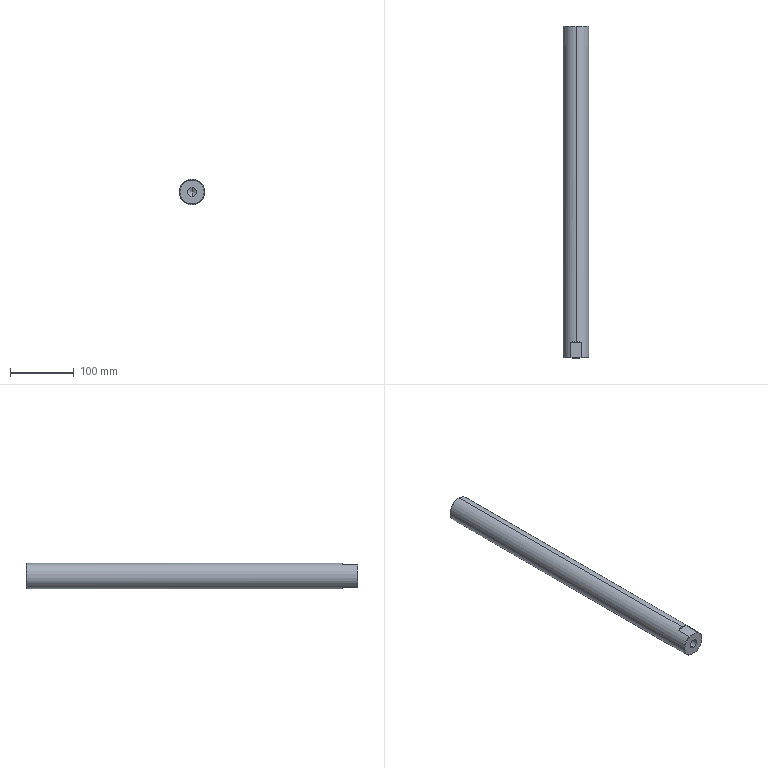Component | SolidWorks | RisingGuidePost-1 | 1 solid | 20 faces | box 40 x 520 x 40 mm | volume 643630 mm3 | cone 8 | cylinder 6 | plane 6 | commonest cylinder face diameters 14 x2 10.2 x2 40 x2
build123d program:
from build123d import *

# Parameters (mm, degrees)
SKETCH1_R              = 20
BOSS_EXTRUDE1_DEPTH    = 260
CHAMFER1_SIZE          = 1
M12_TAPPED_HOLE1_D     = 10.2
M12_TAPPED_HOLE1_DEPTH = 29.25
M12_TAPPED_HOLE1_TIP   = 3.064
M16_TAPPED_HOLE1_D     = 14
M16_TAPPED_HOLE1_DEPTH = 38
M16_TAPPED_HOLE1_TIP   = 4.206
SKETCH6_W              = 59.631
SKETCH6_H              = 15.313
SKETCH6_W_2            = 70.228
SKETCH6_H_2            = 16.123
CUT_EXTRUDE1_DEPTH     = 25


with BuildPart() as part:
    # Sketch1 → Boss-Extrude1 (new, symmetric)
    with BuildSketch(Plane(origin=(0, 0, 0), x_dir=(1, 0, 0), z_dir=(0, 1, 0))):
        with Locations(Location((0, 0, 0), (0, 0, 270))):
            Circle(SKETCH1_R)
    extrude(amount=BOSS_EXTRUDE1_DEPTH, both=True)

    # Chamfer1
    chamfer1_edges = [part.edges().sort_by_distance(p)[0] for p in [
        (0, -260, -20),
        (0, 260, -20),
    ]]
    chamfer(chamfer1_edges, length=CHAMFER1_SIZE)

    # M12 Tapped Hole1
    with Locations(Plane(origin=(0, 260, 0), x_dir=(1, 0, 0), z_dir=(0, 1, 0))):
        with Locations((0, 0)):
            Hole(M12_TAPPED_HOLE1_D / 2, depth=M12_TAPPED_HOLE1_DEPTH)
            with Locations((0, 0, -(M12_TAPPED_HOLE1_DEPTH + M12_TAPPED_HOLE1_TIP / 2))):  # 118° drill point
                Cone(0, M12_TAPPED_HOLE1_D / 2, M12_TAPPED_HOLE1_TIP, mode=Mode.SUBTRACT)

    # M16 Tapped Hole1
    with Locations(Plane(origin=(0, -260, 0), x_dir=(-1, 0, 0), z_dir=(0, -1, 0))):
        with Locations((0, 0)):
            Hole(M16_TAPPED_HOLE1_D / 2, depth=M16_TAPPED_HOLE1_DEPTH)
            with Locations((0, 0, -(M16_TAPPED_HOLE1_DEPTH + M16_TAPPED_HOLE1_TIP / 2))):  # 118° drill point
                Cone(0, M16_TAPPED_HOLE1_D / 2, M16_TAPPED_HOLE1_TIP, mode=Mode.SUBTRACT)

    # Sketch6 → Cut-Extrude1 (cut)
    with BuildSketch(Plane.XZ.offset(260)):
        with Locations((-1.489, 25.656)):
            Rectangle(SKETCH6_W, SKETCH6_H)
        with Locations((-1.031, -26.062)):
            Rectangle(SKETCH6_W_2, SKETCH6_H_2)
    extrude(amount=-CUT_EXTRUDE1_DEPTH, mode=Mode.SUBTRACT)


solid = part.part

# Placed as in the assembly
solid = solid.moved(Location((-194.507, -34.411, 458), (0, 0, 0)))
STEP:
#1=CARTESIAN_POINT('',(-7.658,-10.095,18.307));
#2=VERTEX_POINT('',#1);
#3=CARTESIAN_POINT('',(-7.658,-10.095,17.756));
#4=VERTEX_POINT('',#3);
#5=CARTESIAN_POINT('',(-7.658,-10.095,18.031));
#6=DIRECTION('',(0.,-1.,0.));
#7=DIRECTION('',(0.,0.,-1.));
#8=AXIS2_PLACEMENT_3D('',#5,#6,#7);
#9=CIRCLE('',#8,0.2756);
#10=EDGE_CURVE('',#2,#4,#9,.T.);
#11=ORIENTED_EDGE('',*,*,#10,.F.);
#12=CARTESIAN_POINT('',(-7.658,-11.591,18.307));
#13=VERTEX_POINT('',#12);
#14=CARTESIAN_POINT('',(-7.658,-11.591,18.307));
#15=DIRECTION('',(0.,-1.,0.));
#16=VECTOR('',#15,39.37);
#17=LINE('',#14,#16);
#18=EDGE_CURVE('',#2,#13,#17,.T.);
#19=ORIENTED_EDGE('',*,*,#18,.T.);
#20=CARTESIAN_POINT('',(-7.658,-11.591,17.756));
#21=VERTEX_POINT('',#20);
#22=CARTESIAN_POINT('',(-7.658,-11.591,18.031));
#23=DIRECTION('',(0.,-1.,0.));
#24=DIRECTION('',(0.,0.,-1.));
#25=AXIS2_PLACEMENT_3D('',#22,#23,#24);
#26=CIRCLE('',#25,0.2756);
#27=EDGE_CURVE('',#13,#21,#26,.T.);
#28=ORIENTED_EDGE('',*,*,#27,.T.);
#29=CARTESIAN_POINT('',(-7.658,-11.591,17.756));
#30=DIRECTION('',(0.,-1.,0.));
#31=VECTOR('',#30,39.37);
#32=LINE('',#29,#31);
#33=EDGE_CURVE('',#4,#21,#32,.T.);
#34=ORIENTED_EDGE('',*,*,#33,.F.);
#35=EDGE_LOOP('',(#11,#19,#28,#34));
#36=FACE_OUTER_BOUND('',#35,.T.);
#37=CARTESIAN_POINT('',(-7.658,-11.591,18.031));
#38=DIRECTION('',(0.,-1.,0.));
#39=DIRECTION('',(0.,0.,-1.));
#40=AXIS2_PLACEMENT_3D('',#37,#38,#39);
#41=CYLINDRICAL_SURFACE('',#40,0.2756);
#42=ADVANCED_FACE('',(#36),#41,.F.);
#43=CARTESIAN_POINT('',(-7.658,-9.929,18.031));
#44=VERTEX_POINT('',#43);
#45=CARTESIAN_POINT('',(-7.658,-10.095,17.756));
#46=DIRECTION('',(0.,-0.515,-0.8572));
#47=VECTOR('',#46,39.37);
#48=LINE('',#45,#47);
#49=EDGE_CURVE('',#44,#4,#48,.T.);
#50=ORIENTED_EDGE('',*,*,#49,.F.);
#51=CARTESIAN_POINT('',(-7.658,-10.095,18.307));
#52=DIRECTION('',(0.,-0.515,0.8572));
#53=VECTOR('',#52,39.37);
#54=LINE('',#51,#53);
#55=EDGE_CURVE('',#44,#2,#54,.T.);
#56=ORIENTED_EDGE('',*,*,#55,.T.);
#57=ORIENTED_EDGE('',*,*,#10,.T.);
#58=EDGE_LOOP('',(#50,#56,#57));
#59=FACE_OUTER_BOUND('',#58,.T.);
#60=CARTESIAN_POINT('',(-7.658,-10.095,18.031));
#61=DIRECTION('',(0.,-1.,0.));
#62=DIRECTION('',(0.,0.,-1.));
#63=AXIS2_PLACEMENT_3D('',#60,#61,#62);
#64=CONICAL_SURFACE('',#63,0.2756,1.03);
#65=ADVANCED_FACE('',(#59),#64,.F.);
#66=CARTESIAN_POINT('',(-7.658,7.73,17.831));
#67=VERTEX_POINT('',#66);
#68=CARTESIAN_POINT('',(-7.658,7.73,18.232));
#69=VERTEX_POINT('',#68);
#70=CARTESIAN_POINT('',(-7.658,7.73,18.031));
#71=DIRECTION('',(0.,1.,0.));
#72=DIRECTION('',(0.,0.,1.));
#73=AXIS2_PLACEMENT_3D('',#70,#71,#72);
#74=CIRCLE('',#73,0.2008);
#75=EDGE_CURVE('',#67,#69,#74,.T.);
#76=ORIENTED_EDGE('',*,*,#75,.F.);
#77=CARTESIAN_POINT('',(-7.658,8.881,17.831));
#78=VERTEX_POINT('',#77);
#79=CARTESIAN_POINT('',(-7.658,8.881,17.831));
#80=DIRECTION('',(0.,1.,0.));
#81=VECTOR('',#80,39.37);
#82=LINE('',#79,#81);
#83=EDGE_CURVE('',#67,#78,#82,.T.);
#84=ORIENTED_EDGE('',*,*,#83,.T.);
#85=CARTESIAN_POINT('',(-7.658,8.881,18.232));
#86=VERTEX_POINT('',#85);
#87=CARTESIAN_POINT('',(-7.658,8.881,18.031));
#88=DIRECTION('',(0.,1.,0.));
#89=DIRECTION('',(0.,0.,1.));
#90=AXIS2_PLACEMENT_3D('',#87,#88,#89);
#91=CIRCLE('',#90,0.2008);
#92=EDGE_CURVE('',#78,#86,#91,.T.);
#93=ORIENTED_EDGE('',*,*,#92,.T.);
#94=CARTESIAN_POINT('',(-7.658,8.881,18.232));
#95=DIRECTION('',(0.,1.,0.));
#96=VECTOR('',#95,39.37);
#97=LINE('',#94,#96);
#98=EDGE_CURVE('',#69,#86,#97,.T.);
#99=ORIENTED_EDGE('',*,*,#98,.F.);
#100=EDGE_LOOP('',(#76,#84,#93,#99));
#101=FACE_OUTER_BOUND('',#100,.T.);
#102=CARTESIAN_POINT('',(-7.658,8.881,18.031));
#103=DIRECTION('',(0.,1.,0.));
#104=DIRECTION('',(0.,0.,1.));
#105=AXIS2_PLACEMENT_3D('',#102,#103,#104);
#106=CYLINDRICAL_SURFACE('',#105,0.2008);
#107=ADVANCED_FACE('',(#101),#106,.F.);
#108=CARTESIAN_POINT('',(-7.658,7.609,18.031));
#109=VERTEX_POINT('',#108);
#110=CARTESIAN_POINT('',(-7.658,7.73,18.232));
#111=DIRECTION('',(0.,0.515,0.8572));
#112=VECTOR('',#111,39.37);
#113=LINE('',#110,#112);
#114=EDGE_CURVE('',#109,#69,#113,.T.);
#115=ORIENTED_EDGE('',*,*,#114,.F.);
#116=CARTESIAN_POINT('',(-7.658,7.73,17.831));
#117=DIRECTION('',(0.,0.515,-0.8572));
#118=VECTOR('',#117,39.37);
#119=LINE('',#116,#118);
#120=EDGE_CURVE('',#109,#67,#119,.T.);
#121=ORIENTED_EDGE('',*,*,#120,.T.);
#122=ORIENTED_EDGE('',*,*,#75,.T.);
#123=EDGE_LOOP('',(#115,#121,#122));
#124=FACE_OUTER_BOUND('',#123,.T.);
#125=CARTESIAN_POINT('',(-7.658,7.73,18.031));
#126=DIRECTION('',(0.,1.,0.));
#127=DIRECTION('',(0.,0.,1.));
#128=AXIS2_PLACEMENT_3D('',#125,#126,#127);
#129=CONICAL_SURFACE('',#128,0.2008,1.03);
#130=ADVANCED_FACE('',(#124),#129,.F.);
#131=CARTESIAN_POINT('',(-7.658,8.881,18.78));
#132=VERTEX_POINT('',#131);
#133=CARTESIAN_POINT('',(-7.658,8.881,17.283));
#134=VERTEX_POINT('',#133);
#135=CARTESIAN_POINT('',(-7.658,8.881,18.031));
#136=DIRECTION('',(0.,1.,0.));
#137=DIRECTION('',(0.,0.,1.));
#138=AXIS2_PLACEMENT_3D('',#135,#136,#137);
#139=CIRCLE('',#138,0.748);
#140=EDGE_CURVE('',#132,#134,#139,.T.);
#141=ORIENTED_EDGE('',*,*,#140,.F.);
#142=CARTESIAN_POINT('',(-7.658,8.842,18.819));
#143=VERTEX_POINT('',#142);
#144=CARTESIAN_POINT('',(-7.658,8.881,18.78));
#145=DIRECTION('',(0.,-0.7071,0.7071));
#146=VECTOR('',#145,39.37);
#147=LINE('',#144,#146);
#148=EDGE_CURVE('',#132,#143,#147,.T.);
#149=ORIENTED_EDGE('',*,*,#148,.T.);
#150=CARTESIAN_POINT('',(-7.658,8.842,17.244));
#151=VERTEX_POINT('',#150);
#152=CARTESIAN_POINT('',(-7.658,8.842,18.031));
#153=DIRECTION('',(0.,-1.,0.));
#154=DIRECTION('',(0.,0.,1.));
#155=AXIS2_PLACEMENT_3D('',#152,#153,#154);
#156=CIRCLE('',#155,0.7874);
#157=EDGE_CURVE('',#151,#143,#156,.T.);
#158=ORIENTED_EDGE('',*,*,#157,.F.);
#159=CARTESIAN_POINT('',(-7.658,8.881,17.283));
#160=DIRECTION('',(0.,-0.7071,-0.7071));
#161=VECTOR('',#160,39.37);
#162=LINE('',#159,#161);
#163=EDGE_CURVE('',#134,#151,#162,.T.);
#164=ORIENTED_EDGE('',*,*,#163,.F.);
#165=EDGE_LOOP('',(#141,#149,#158,#164));
#166=FACE_OUTER_BOUND('',#165,.T.);
#167=CARTESIAN_POINT('',(-7.658,8.881,18.031));
#168=DIRECTION('',(0.,-1.,0.));
#169=DIRECTION('',(0.,0.,-1.));
#170=AXIS2_PLACEMENT_3D('',#167,#168,#169);
#171=CONICAL_SURFACE('',#170,0.748,0.7854);
#172=ADVANCED_FACE('',(#166),#171,.T.);
#173=ORIENTED_EDGE('',*,*,#157,.T.);
#174=CARTESIAN_POINT('',(-7.658,-10.607,18.819));
#175=VERTEX_POINT('',#174);
#176=CARTESIAN_POINT('',(-7.658,8.881,18.819));
#177=DIRECTION('',(0.,-1.,0.));
#178=VECTOR('',#177,39.37);
#179=LINE('',#176,#178);
#180=EDGE_CURVE('',#143,#175,#179,.T.);
#181=ORIENTED_EDGE('',*,*,#180,.T.);
#182=CARTESIAN_POINT('',(-7.315,-10.607,18.74));
#183=VERTEX_POINT('',#182);
#184=CARTESIAN_POINT('',(-7.658,-10.607,18.031));
#185=DIRECTION('',(0.,-1.,0.));
#186=DIRECTION('',(0.,0.,-1.));
#187=AXIS2_PLACEMENT_3D('',#184,#185,#186);
#188=CIRCLE('',#187,0.7874);
#189=EDGE_CURVE('',#183,#175,#188,.T.);
#190=ORIENTED_EDGE('',*,*,#189,.F.);
#191=CARTESIAN_POINT('',(-7.315,-11.552,18.74));
#192=VERTEX_POINT('',#191);
#193=CARTESIAN_POINT('',(-7.315,8.881,18.74));
#194=DIRECTION('',(0.,-1.,0.));
#195=VECTOR('',#194,39.37);
#196=LINE('',#193,#195);
#197=EDGE_CURVE('',#183,#192,#196,.T.);
#198=ORIENTED_EDGE('',*,*,#197,.T.);
#199=CARTESIAN_POINT('',(-7.315,-11.552,17.323));
#200=VERTEX_POINT('',#199);
#201=CARTESIAN_POINT('',(-7.658,-11.552,18.031));
#202=DIRECTION('',(0.,1.,0.));
#203=DIRECTION('',(0.,0.,1.));
#204=AXIS2_PLACEMENT_3D('',#201,#202,#203);
#205=CIRCLE('',#204,0.7874);
#206=EDGE_CURVE('',#192,#200,#205,.T.);
#207=ORIENTED_EDGE('',*,*,#206,.T.);
#208=CARTESIAN_POINT('',(-7.315,-10.607,17.323));
#209=VERTEX_POINT('',#208);
#210=CARTESIAN_POINT('',(-7.315,8.881,17.323));
#211=DIRECTION('',(0.,1.,0.));
#212=VECTOR('',#211,39.37);
#213=LINE('',#210,#212);
#214=EDGE_CURVE('',#200,#209,#213,.T.);
#215=ORIENTED_EDGE('',*,*,#214,.T.);
#216=CARTESIAN_POINT('',(-7.658,-10.607,17.244));
#217=VERTEX_POINT('',#216);
#218=CARTESIAN_POINT('',(-7.658,-10.607,18.031));
#219=DIRECTION('',(0.,1.,0.));
#220=DIRECTION('',(0.,0.,1.));
#221=AXIS2_PLACEMENT_3D('',#218,#219,#220);
#222=CIRCLE('',#221,0.7874);
#223=EDGE_CURVE('',#209,#217,#222,.T.);
#224=ORIENTED_EDGE('',*,*,#223,.T.);
#225=CARTESIAN_POINT('',(-7.658,8.881,17.244));
#226=DIRECTION('',(0.,-1.,0.));
#227=VECTOR('',#226,39.37);
#228=LINE('',#225,#227);
#229=EDGE_CURVE('',#151,#217,#228,.T.);
#230=ORIENTED_EDGE('',*,*,#229,.F.);
#231=EDGE_LOOP('',(#173,#181,#190,#198,#207,#215,#224,#230));
#232=FACE_OUTER_BOUND('',#231,.T.);
#233=CARTESIAN_POINT('',(-7.658,8.881,18.031));
#234=DIRECTION('',(0.,-1.,0.));
#235=DIRECTION('',(0.,0.,-1.));
#236=AXIS2_PLACEMENT_3D('',#233,#234,#235);
#237=CYLINDRICAL_SURFACE('',#236,0.7874);
#238=ADVANCED_FACE('',(#232),#237,.T.);
#239=CARTESIAN_POINT('',(-7.418,-11.591,17.323));
#240=VERTEX_POINT('',#239);
#241=CARTESIAN_POINT('',(-7.315,-11.552,17.323));
#242=CARTESIAN_POINT('',(-7.348,-11.566,17.323));
#243=CARTESIAN_POINT('',(-7.383,-11.58,17.323));
#244=CARTESIAN_POINT('',(-7.418,-11.591,17.323));
#245=B_SPLINE_CURVE_WITH_KNOTS('',3,(#241,#242,#243,#244),.UNSPECIFIED.,.F.,.F.,(4,4),(0.03971,0.04253),.UNSPECIFIED.);
#246=EDGE_CURVE('',#200,#240,#245,.T.);
#247=ORIENTED_EDGE('',*,*,#246,.F.);
#248=ORIENTED_EDGE('',*,*,#206,.F.);
#249=CARTESIAN_POINT('',(-7.418,-11.591,18.74));
#250=VERTEX_POINT('',#249);
#251=CARTESIAN_POINT('',(-7.418,-11.591,18.74));
#252=CARTESIAN_POINT('',(-7.383,-11.58,18.74));
#253=CARTESIAN_POINT('',(-7.348,-11.566,18.74));
#254=CARTESIAN_POINT('',(-7.315,-11.552,18.74));
#255=B_SPLINE_CURVE_WITH_KNOTS('',3,(#251,#252,#253,#254),.UNSPECIFIED.,.F.,.F.,(4,4),(0.0549,0.05771),.UNSPECIFIED.);
#256=EDGE_CURVE('',#250,#192,#255,.T.);
#257=ORIENTED_EDGE('',*,*,#256,.F.);
#258=CARTESIAN_POINT('',(-7.658,-11.591,18.031));
#259=DIRECTION('',(0.,-1.,0.));
#260=DIRECTION('',(0.,0.,1.));
#261=AXIS2_PLACEMENT_3D('',#258,#259,#260);
#262=CIRCLE('',#261,0.748);
#263=EDGE_CURVE('',#240,#250,#262,.T.);
#264=ORIENTED_EDGE('',*,*,#263,.F.);
#265=EDGE_LOOP('',(#247,#248,#257,#264));
#266=FACE_OUTER_BOUND('',#265,.T.);
#267=CARTESIAN_POINT('',(-7.658,-11.552,18.031));
#268=DIRECTION('',(0.,1.,0.));
#269=DIRECTION('',(0.,0.,1.));
#270=AXIS2_PLACEMENT_3D('',#267,#268,#269);
#271=CONICAL_SURFACE('',#270,0.7874,0.7854);
#272=ADVANCED_FACE('',(#266),#271,.T.);
#273=ORIENTED_EDGE('',*,*,#180,.F.);
#274=CARTESIAN_POINT('',(-7.658,8.842,18.031));
#275=DIRECTION('',(0.,-1.,0.));
#276=DIRECTION('',(0.,0.,1.));
#277=AXIS2_PLACEMENT_3D('',#274,#275,#276);
#278=CIRCLE('',#277,0.7874);
#279=EDGE_CURVE('',#143,#151,#278,.T.);
#280=ORIENTED_EDGE('',*,*,#279,.T.);
#281=ORIENTED_EDGE('',*,*,#229,.T.);
#282=CARTESIAN_POINT('',(-8.001,-10.607,17.323));
#283=VERTEX_POINT('',#282);
#284=CARTESIAN_POINT('',(-7.658,-10.607,18.031));
#285=DIRECTION('',(0.,1.,0.));
#286=DIRECTION('',(0.,0.,1.));
#287=AXIS2_PLACEMENT_3D('',#284,#285,#286);
#288=CIRCLE('',#287,0.7874);
#289=EDGE_CURVE('',#217,#283,#288,.T.);
#290=ORIENTED_EDGE('',*,*,#289,.T.);
#291=CARTESIAN_POINT('',(-8.001,-11.552,17.323));
#292=VERTEX_POINT('',#291);
#293=CARTESIAN_POINT('',(-8.001,8.881,17.323));
#294=DIRECTION('',(0.,-1.,0.));
#295=VECTOR('',#294,39.37);
#296=LINE('',#293,#295);
#297=EDGE_CURVE('',#283,#292,#296,.T.);
#298=ORIENTED_EDGE('',*,*,#297,.T.);
#299=CARTESIAN_POINT('',(-8.001,-11.552,18.74));
#300=VERTEX_POINT('',#299);
#301=CARTESIAN_POINT('',(-7.658,-11.552,18.031));
#302=DIRECTION('',(0.,1.,0.));
#303=DIRECTION('',(0.,0.,1.));
#304=AXIS2_PLACEMENT_3D('',#301,#302,#303);
#305=CIRCLE('',#304,0.7874);
#306=EDGE_CURVE('',#292,#300,#305,.T.);
#307=ORIENTED_EDGE('',*,*,#306,.T.);
#308=CARTESIAN_POINT('',(-8.001,-10.607,18.74));
#309=VERTEX_POINT('',#308);
#310=CARTESIAN_POINT('',(-8.001,8.881,18.74));
#311=DIRECTION('',(0.,1.,0.));
#312=VECTOR('',#311,39.37);
#313=LINE('',#310,#312);
#314=EDGE_CURVE('',#300,#309,#313,.T.);
#315=ORIENTED_EDGE('',*,*,#314,.T.);
#316=CARTESIAN_POINT('',(-7.658,-10.607,18.031));
#317=DIRECTION('',(0.,-1.,0.));
#318=DIRECTION('',(0.,0.,-1.));
#319=AXIS2_PLACEMENT_3D('',#316,#317,#318);
#320=CIRCLE('',#319,0.7874);
#321=EDGE_CURVE('',#175,#309,#320,.T.);
#322=ORIENTED_EDGE('',*,*,#321,.F.);
#323=EDGE_LOOP('',(#273,#280,#281,#290,#298,#307,#315,#322));
#324=FACE_OUTER_BOUND('',#323,.T.);
#325=CARTESIAN_POINT('',(-7.658,8.881,18.031));
#326=DIRECTION('',(0.,-1.,0.));
#327=DIRECTION('',(0.,0.,-1.));
#328=AXIS2_PLACEMENT_3D('',#325,#326,#327);
#329=CYLINDRICAL_SURFACE('',#328,0.7874);
#330=ADVANCED_FACE('',(#324),#329,.T.);
#331=CARTESIAN_POINT('',(-7.658,8.881,18.031));
#332=DIRECTION('',(0.,1.,0.));
#333=DIRECTION('',(0.,0.,1.));
#334=AXIS2_PLACEMENT_3D('',#331,#332,#333);
#335=CIRCLE('',#334,0.2008);
#336=EDGE_CURVE('',#86,#78,#335,.T.);
#337=ORIENTED_EDGE('',*,*,#336,.F.);
#338=ORIENTED_EDGE('',*,*,#92,.F.);
#339=EDGE_LOOP('',(#337,#338));
#340=FACE_BOUND('',#339,.T.);
#341=CARTESIAN_POINT('',(-7.658,8.881,18.031));
#342=DIRECTION('',(0.,1.,0.));
#343=DIRECTION('',(0.,0.,1.));
#344=AXIS2_PLACEMENT_3D('',#341,#342,#343);
#345=CIRCLE('',#344,0.748);
#346=EDGE_CURVE('',#134,#132,#345,.T.);
#347=ORIENTED_EDGE('',*,*,#346,.T.);
#348=ORIENTED_EDGE('',*,*,#140,.T.);
#349=EDGE_LOOP('',(#347,#348));
#350=FACE_OUTER_BOUND('',#349,.T.);
#351=CARTESIAN_POINT('',(-7.658,8.881,18.031));
#352=DIRECTION('',(0.,1.,0.));
#353=DIRECTION('',(0.,0.,1.));
#354=AXIS2_PLACEMENT_3D('',#351,#352,#353);
#355=PLANE('',#354);
#356=ADVANCED_FACE('',(#340,#350),#355,.T.);
#357=CARTESIAN_POINT('',(-7.658,-11.591,18.031));
#358=DIRECTION('',(0.,-1.,0.));
#359=DIRECTION('',(0.,0.,-1.));
#360=AXIS2_PLACEMENT_3D('',#357,#358,#359);
#361=CIRCLE('',#360,0.2756);
#362=EDGE_CURVE('',#21,#13,#361,.T.);
#363=ORIENTED_EDGE('',*,*,#362,.F.);
#364=ORIENTED_EDGE('',*,*,#27,.F.);
#365=EDGE_LOOP('',(#363,#364));
#366=FACE_BOUND('',#365,.T.);
#367=CARTESIAN_POINT('',(-7.897,-11.591,18.74));
#368=VERTEX_POINT('',#367);
#369=CARTESIAN_POINT('',(-7.897,-11.591,17.323));
#370=VERTEX_POINT('',#369);
#371=CARTESIAN_POINT('',(-7.658,-11.591,18.031));
#372=DIRECTION('',(0.,-1.,0.));
#373=DIRECTION('',(-0.,0.,1.));
#374=AXIS2_PLACEMENT_3D('',#371,#372,#373);
#375=CIRCLE('',#374,0.748);
#376=EDGE_CURVE('',#368,#370,#375,.T.);
#377=ORIENTED_EDGE('',*,*,#376,.T.);
#378=CARTESIAN_POINT('',(-9.081,-11.591,17.323));
#379=DIRECTION('',(-1.,0.,0.));
#380=VECTOR('',#379,39.37);
#381=LINE('',#378,#380);
#382=EDGE_CURVE('',#240,#370,#381,.T.);
#383=ORIENTED_EDGE('',*,*,#382,.F.);
#384=ORIENTED_EDGE('',*,*,#263,.T.);
#385=CARTESIAN_POINT('',(-8.89,-11.591,18.74));
#386=DIRECTION('',(1.,0.,0.));
#387=VECTOR('',#386,39.37);
#388=LINE('',#385,#387);
#389=EDGE_CURVE('',#368,#250,#388,.T.);
#390=ORIENTED_EDGE('',*,*,#389,.F.);
#391=EDGE_LOOP('',(#377,#383,#384,#390));
#392=FACE_OUTER_BOUND('',#391,.T.);
#393=CARTESIAN_POINT('',(-7.658,-11.591,18.031));
#394=DIRECTION('',(0.,1.,0.));
#395=DIRECTION('',(0.,0.,1.));
#396=AXIS2_PLACEMENT_3D('',#393,#394,#395);
#397=PLANE('',#396);
#398=ADVANCED_FACE('',(#366,#392),#397,.F.);
#399=ORIENTED_EDGE('',*,*,#148,.F.);
#400=ORIENTED_EDGE('',*,*,#346,.F.);
#401=ORIENTED_EDGE('',*,*,#163,.T.);
#402=ORIENTED_EDGE('',*,*,#279,.F.);
#403=EDGE_LOOP('',(#399,#400,#401,#402));
#404=FACE_OUTER_BOUND('',#403,.T.);
#405=CARTESIAN_POINT('',(-7.658,8.881,18.031));
#406=DIRECTION('',(0.,-1.,0.));
#407=DIRECTION('',(0.,0.,-1.));
#408=AXIS2_PLACEMENT_3D('',#405,#406,#407);
#409=CONICAL_SURFACE('',#408,0.748,0.7854);
#410=ADVANCED_FACE('',(#404),#409,.T.);
#411=CARTESIAN_POINT('',(-7.897,-11.591,17.323));
#412=CARTESIAN_POINT('',(-7.932,-11.58,17.323));
#413=CARTESIAN_POINT('',(-7.967,-11.566,17.323));
#414=CARTESIAN_POINT('',(-8.001,-11.552,17.323));
#415=B_SPLINE_CURVE_WITH_KNOTS('',3,(#411,#412,#413,#414),.UNSPECIFIED.,.F.,.F.,(4,4),(0.0549,0.05771),.UNSPECIFIED.);
#416=EDGE_CURVE('',#370,#292,#415,.T.);
#417=ORIENTED_EDGE('',*,*,#416,.F.);
#418=ORIENTED_EDGE('',*,*,#376,.F.);
#419=CARTESIAN_POINT('',(-8.001,-11.552,18.74));
#420=CARTESIAN_POINT('',(-7.967,-11.566,18.74));
#421=CARTESIAN_POINT('',(-7.933,-11.58,18.74));
#422=CARTESIAN_POINT('',(-7.897,-11.591,18.74));
#423=B_SPLINE_CURVE_WITH_KNOTS('',3,(#419,#420,#421,#422),.UNSPECIFIED.,.F.,.F.,(4,4),(0.03971,0.04253),.UNSPECIFIED.);
#424=EDGE_CURVE('',#300,#368,#423,.T.);
#425=ORIENTED_EDGE('',*,*,#424,.F.);
#426=ORIENTED_EDGE('',*,*,#306,.F.);
#427=EDGE_LOOP('',(#417,#418,#425,#426));
#428=FACE_OUTER_BOUND('',#427,.T.);
#429=CARTESIAN_POINT('',(-7.658,-11.552,18.031));
#430=DIRECTION('',(0.,1.,0.));
#431=DIRECTION('',(0.,0.,1.));
#432=AXIS2_PLACEMENT_3D('',#429,#430,#431);
#433=CONICAL_SURFACE('',#432,0.7874,0.7854);
#434=ADVANCED_FACE('',(#428),#433,.T.);
#435=ORIENTED_EDGE('',*,*,#120,.F.);
#436=ORIENTED_EDGE('',*,*,#114,.T.);
#437=CARTESIAN_POINT('',(-7.658,7.73,18.031));
#438=DIRECTION('',(0.,1.,0.));
#439=DIRECTION('',(0.,0.,1.));
#440=AXIS2_PLACEMENT_3D('',#437,#438,#439);
#441=CIRCLE('',#440,0.2008);
#442=EDGE_CURVE('',#69,#67,#441,.T.);
#443=ORIENTED_EDGE('',*,*,#442,.T.);
#444=EDGE_LOOP('',(#435,#436,#443));
#445=FACE_OUTER_BOUND('',#444,.T.);
#446=CARTESIAN_POINT('',(-7.658,7.73,18.031));
#447=DIRECTION('',(0.,1.,0.));
#448=DIRECTION('',(0.,0.,1.));
#449=AXIS2_PLACEMENT_3D('',#446,#447,#448);
#450=CONICAL_SURFACE('',#449,0.2008,1.03);
#451=ADVANCED_FACE('',(#445),#450,.F.);
#452=ORIENTED_EDGE('',*,*,#83,.F.);
#453=ORIENTED_EDGE('',*,*,#442,.F.);
#454=ORIENTED_EDGE('',*,*,#98,.T.);
#455=ORIENTED_EDGE('',*,*,#336,.T.);
#456=EDGE_LOOP('',(#452,#453,#454,#455));
#457=FACE_OUTER_BOUND('',#456,.T.);
#458=CARTESIAN_POINT('',(-7.658,8.881,18.031));
#459=DIRECTION('',(0.,1.,0.));
#460=DIRECTION('',(0.,0.,1.));
#461=AXIS2_PLACEMENT_3D('',#458,#459,#460);
#462=CYLINDRICAL_SURFACE('',#461,0.2008);
#463=ADVANCED_FACE('',(#457),#462,.F.);
#464=ORIENTED_EDGE('',*,*,#55,.F.);
#465=ORIENTED_EDGE('',*,*,#49,.T.);
#466=CARTESIAN_POINT('',(-7.658,-10.095,18.031));
#467=DIRECTION('',(0.,-1.,0.));
#468=DIRECTION('',(0.,0.,-1.));
#469=AXIS2_PLACEMENT_3D('',#466,#467,#468);
#470=CIRCLE('',#469,0.2756);
#471=EDGE_CURVE('',#4,#2,#470,.T.);
#472=ORIENTED_EDGE('',*,*,#471,.T.);
#473=EDGE_LOOP('',(#464,#465,#472));
#474=FACE_OUTER_BOUND('',#473,.T.);
#475=CARTESIAN_POINT('',(-7.658,-10.095,18.031));
#476=DIRECTION('',(0.,-1.,0.));
#477=DIRECTION('',(0.,0.,-1.));
#478=AXIS2_PLACEMENT_3D('',#475,#476,#477);
#479=CONICAL_SURFACE('',#478,0.2756,1.03);
#480=ADVANCED_FACE('',(#474),#479,.F.);
#481=ORIENTED_EDGE('',*,*,#18,.F.);
#482=ORIENTED_EDGE('',*,*,#471,.F.);
#483=ORIENTED_EDGE('',*,*,#33,.T.);
#484=ORIENTED_EDGE('',*,*,#362,.T.);
#485=EDGE_LOOP('',(#481,#482,#483,#484));
#486=FACE_OUTER_BOUND('',#485,.T.);
#487=CARTESIAN_POINT('',(-7.658,-11.591,18.031));
#488=DIRECTION('',(0.,-1.,0.));
#489=DIRECTION('',(0.,0.,-1.));
#490=AXIS2_PLACEMENT_3D('',#487,#488,#489);
#491=CYLINDRICAL_SURFACE('',#490,0.2756);
#492=ADVANCED_FACE('',(#486),#491,.F.);
#493=ORIENTED_EDGE('',*,*,#189,.T.);
#494=ORIENTED_EDGE('',*,*,#321,.T.);
#495=CARTESIAN_POINT('',(-8.89,-10.607,18.74));
#496=DIRECTION('',(1.,0.,0.));
#497=VECTOR('',#496,39.37);
#498=LINE('',#495,#497);
#499=EDGE_CURVE('',#309,#183,#498,.T.);
#500=ORIENTED_EDGE('',*,*,#499,.T.);
#501=EDGE_LOOP('',(#493,#494,#500));
#502=FACE_OUTER_BOUND('',#501,.T.);
#503=CARTESIAN_POINT('',(-7.658,-10.607,18.031));
#504=DIRECTION('',(0.,-1.,0.));
#505=DIRECTION('',(0.,0.,-1.));
#506=AXIS2_PLACEMENT_3D('',#503,#504,#505);
#507=PLANE('',#506);
#508=ADVANCED_FACE('',(#502),#507,.T.);
#509=ORIENTED_EDGE('',*,*,#424,.T.);
#510=ORIENTED_EDGE('',*,*,#389,.T.);
#511=ORIENTED_EDGE('',*,*,#256,.T.);
#512=ORIENTED_EDGE('',*,*,#197,.F.);
#513=ORIENTED_EDGE('',*,*,#499,.F.);
#514=ORIENTED_EDGE('',*,*,#314,.F.);
#515=EDGE_LOOP('',(#509,#510,#511,#512,#513,#514));
#516=FACE_OUTER_BOUND('',#515,.T.);
#517=CARTESIAN_POINT('',(-8.89,-10.607,18.74));
#518=DIRECTION('',(0.,0.,-1.));
#519=DIRECTION('',(-1.,0.,0.));
#520=AXIS2_PLACEMENT_3D('',#517,#518,#519);
#521=PLANE('',#520);
#522=ADVANCED_FACE('',(#516),#521,.F.);
#523=CARTESIAN_POINT('',(-9.081,-10.607,17.323));
#524=DIRECTION('',(-1.,0.,0.));
#525=VECTOR('',#524,39.37);
#526=LINE('',#523,#525);
#527=EDGE_CURVE('',#209,#283,#526,.T.);
#528=ORIENTED_EDGE('',*,*,#527,.T.);
#529=ORIENTED_EDGE('',*,*,#289,.F.);
#530=ORIENTED_EDGE('',*,*,#223,.F.);
#531=EDGE_LOOP('',(#528,#529,#530));
#532=FACE_OUTER_BOUND('',#531,.T.);
#533=CARTESIAN_POINT('',(-7.658,-10.607,18.031));
#534=DIRECTION('',(0.,1.,0.));
#535=DIRECTION('',(0.,0.,1.));
#536=AXIS2_PLACEMENT_3D('',#533,#534,#535);
#537=PLANE('',#536);
#538=ADVANCED_FACE('',(#532),#537,.F.);
#539=ORIENTED_EDGE('',*,*,#246,.T.);
#540=ORIENTED_EDGE('',*,*,#382,.T.);
#541=ORIENTED_EDGE('',*,*,#416,.T.);
#542=ORIENTED_EDGE('',*,*,#297,.F.);
#543=ORIENTED_EDGE('',*,*,#527,.F.);
#544=ORIENTED_EDGE('',*,*,#214,.F.);
#545=EDGE_LOOP('',(#539,#540,#541,#542,#543,#544));
#546=FACE_OUTER_BOUND('',#545,.T.);
#547=CARTESIAN_POINT('',(-9.081,-10.607,17.323));
#548=DIRECTION('',(0.,0.,1.));
#549=DIRECTION('',(1.,0.,0.));
#550=AXIS2_PLACEMENT_3D('',#547,#548,#549);
#551=PLANE('',#550);
#552=ADVANCED_FACE('',(#546),#551,.F.);
#553=CLOSED_SHELL('',(#42,#65,#107,#130,#172,#238,#272,#330,#356,#398,#410,#434,#451,#463,#480,#492,#508,#522,#538,#552));
#554=MANIFOLD_SOLID_BREP('',#553);
#555=CARTESIAN_POINT('',(0.,0.,0.));
#556=DIRECTION('',(0.,0.,1.));
#557=DIRECTION('',(1.,0.,0.));
#558=AXIS2_PLACEMENT_3D('',#555,#556,#557);
#559=(LENGTH_UNIT()NAMED_UNIT(*)SI_UNIT($,.METRE.));
#560=LENGTH_MEASURE_WITH_UNIT(LENGTH_MEASURE(0.0254),#559);
#561=DIMENSIONAL_EXPONENTS(1.,0.,0.,0.,0.,0.,0.);
#562=(CONVERSION_BASED_UNIT('',#560)LENGTH_UNIT()NAMED_UNIT(#561));
#563=UNCERTAINTY_MEASURE_WITH_UNIT(LENGTH_MEASURE(0.00001),#562,'','');
#564=(NAMED_UNIT(*)PLANE_ANGLE_UNIT()SI_UNIT($,.RADIAN.));
#565=(NAMED_UNIT(*)SI_UNIT($,.STERADIAN.)SOLID_ANGLE_UNIT());
#566=(GEOMETRIC_REPRESENTATION_CONTEXT(3)GLOBAL_UNCERTAINTY_ASSIGNED_CONTEXT((#563))GLOBAL_UNIT_ASSIGNED_CONTEXT((#562,#564,#565))REPRESENTATION_CONTEXT('',''));
#567=ADVANCED_BREP_SHAPE_REPRESENTATION('',(#554,#558),#566);
#568=COLOUR_RGB('',0.7922,0.8196,0.9333);
#569=FILL_AREA_STYLE_COLOUR('',#568);
#570=FILL_AREA_STYLE('',(#569));
#571=SURFACE_STYLE_FILL_AREA(#570);
#572=SURFACE_SIDE_STYLE('',(#571));
#573=SURFACE_STYLE_USAGE(.BOTH.,#572);
#574=PRESENTATION_STYLE_ASSIGNMENT((#573));
#575=STYLED_ITEM('',(#574),#554);
#576=(LENGTH_UNIT()NAMED_UNIT(*)SI_UNIT($,.METRE.));
#577=LENGTH_MEASURE_WITH_UNIT(LENGTH_MEASURE(0.0254),#576);
#578=DIMENSIONAL_EXPONENTS(1.,0.,0.,0.,0.,0.,0.);
#579=(CONVERSION_BASED_UNIT('',#577)LENGTH_UNIT()NAMED_UNIT(#578));
#580=UNCERTAINTY_MEASURE_WITH_UNIT(LENGTH_MEASURE(0.00001),#579,'','');
#581=(NAMED_UNIT(*)PLANE_ANGLE_UNIT()SI_UNIT($,.RADIAN.));
#582=(NAMED_UNIT(*)SI_UNIT($,.STERADIAN.)SOLID_ANGLE_UNIT());
#583=(GEOMETRIC_REPRESENTATION_CONTEXT(3)GLOBAL_UNCERTAINTY_ASSIGNED_CONTEXT((#580))GLOBAL_UNIT_ASSIGNED_CONTEXT((#579,#581,#582))REPRESENTATION_CONTEXT('',''));
#584=MECHANICAL_DESIGN_GEOMETRIC_PRESENTATION_REPRESENTATION('',(#575),#583);
#585=PRESENTATION_LAYER_ASSIGNMENT('','',(#575));